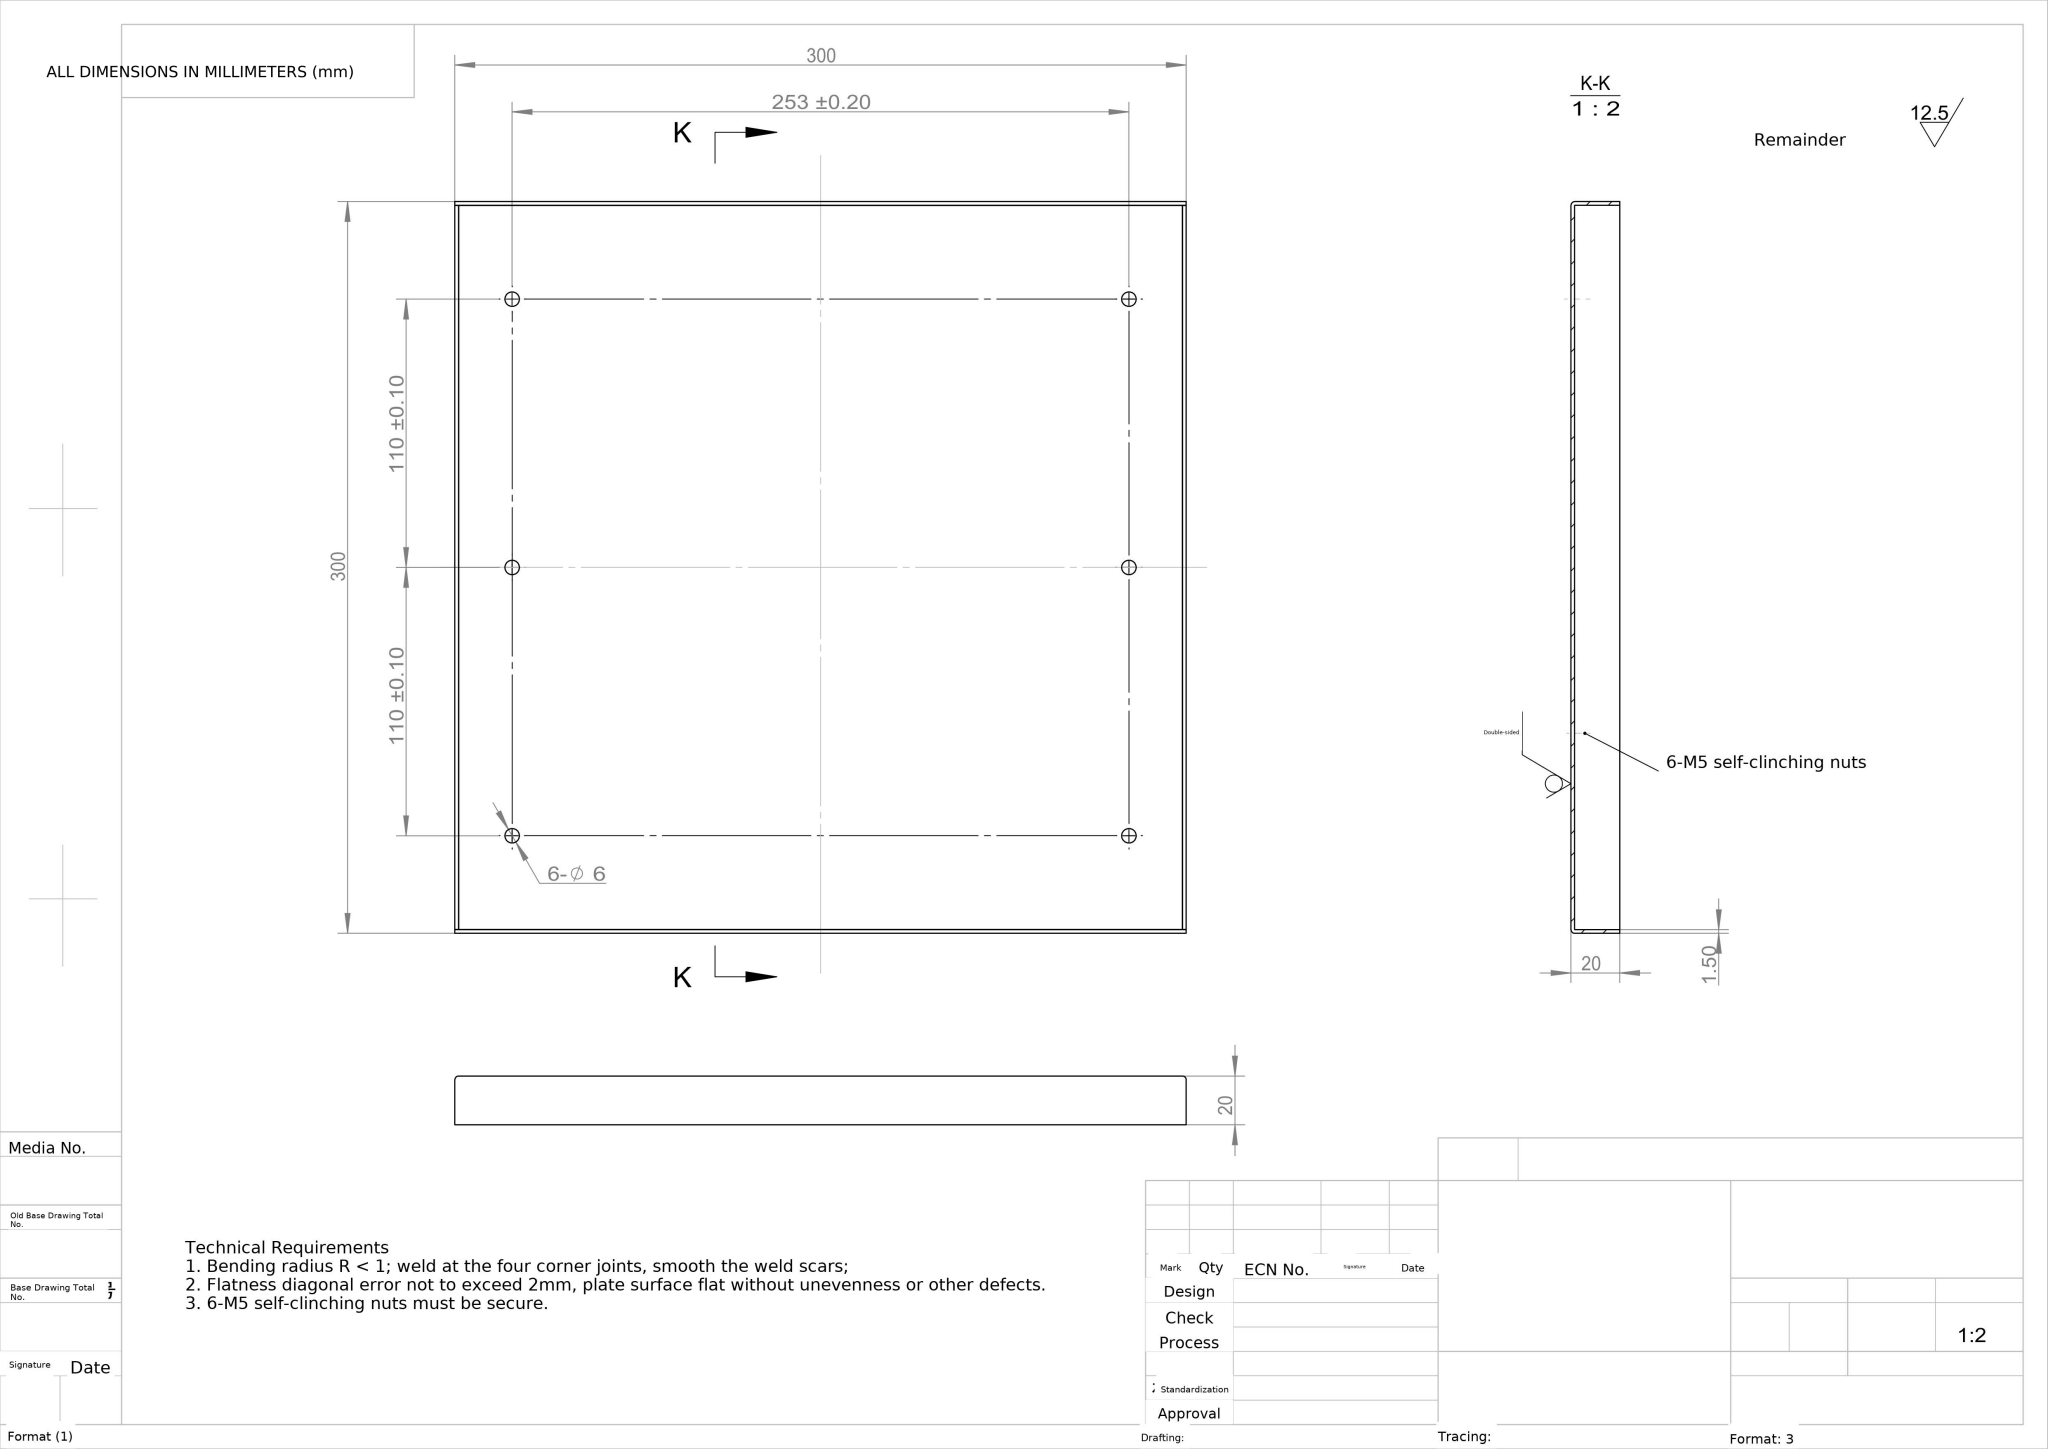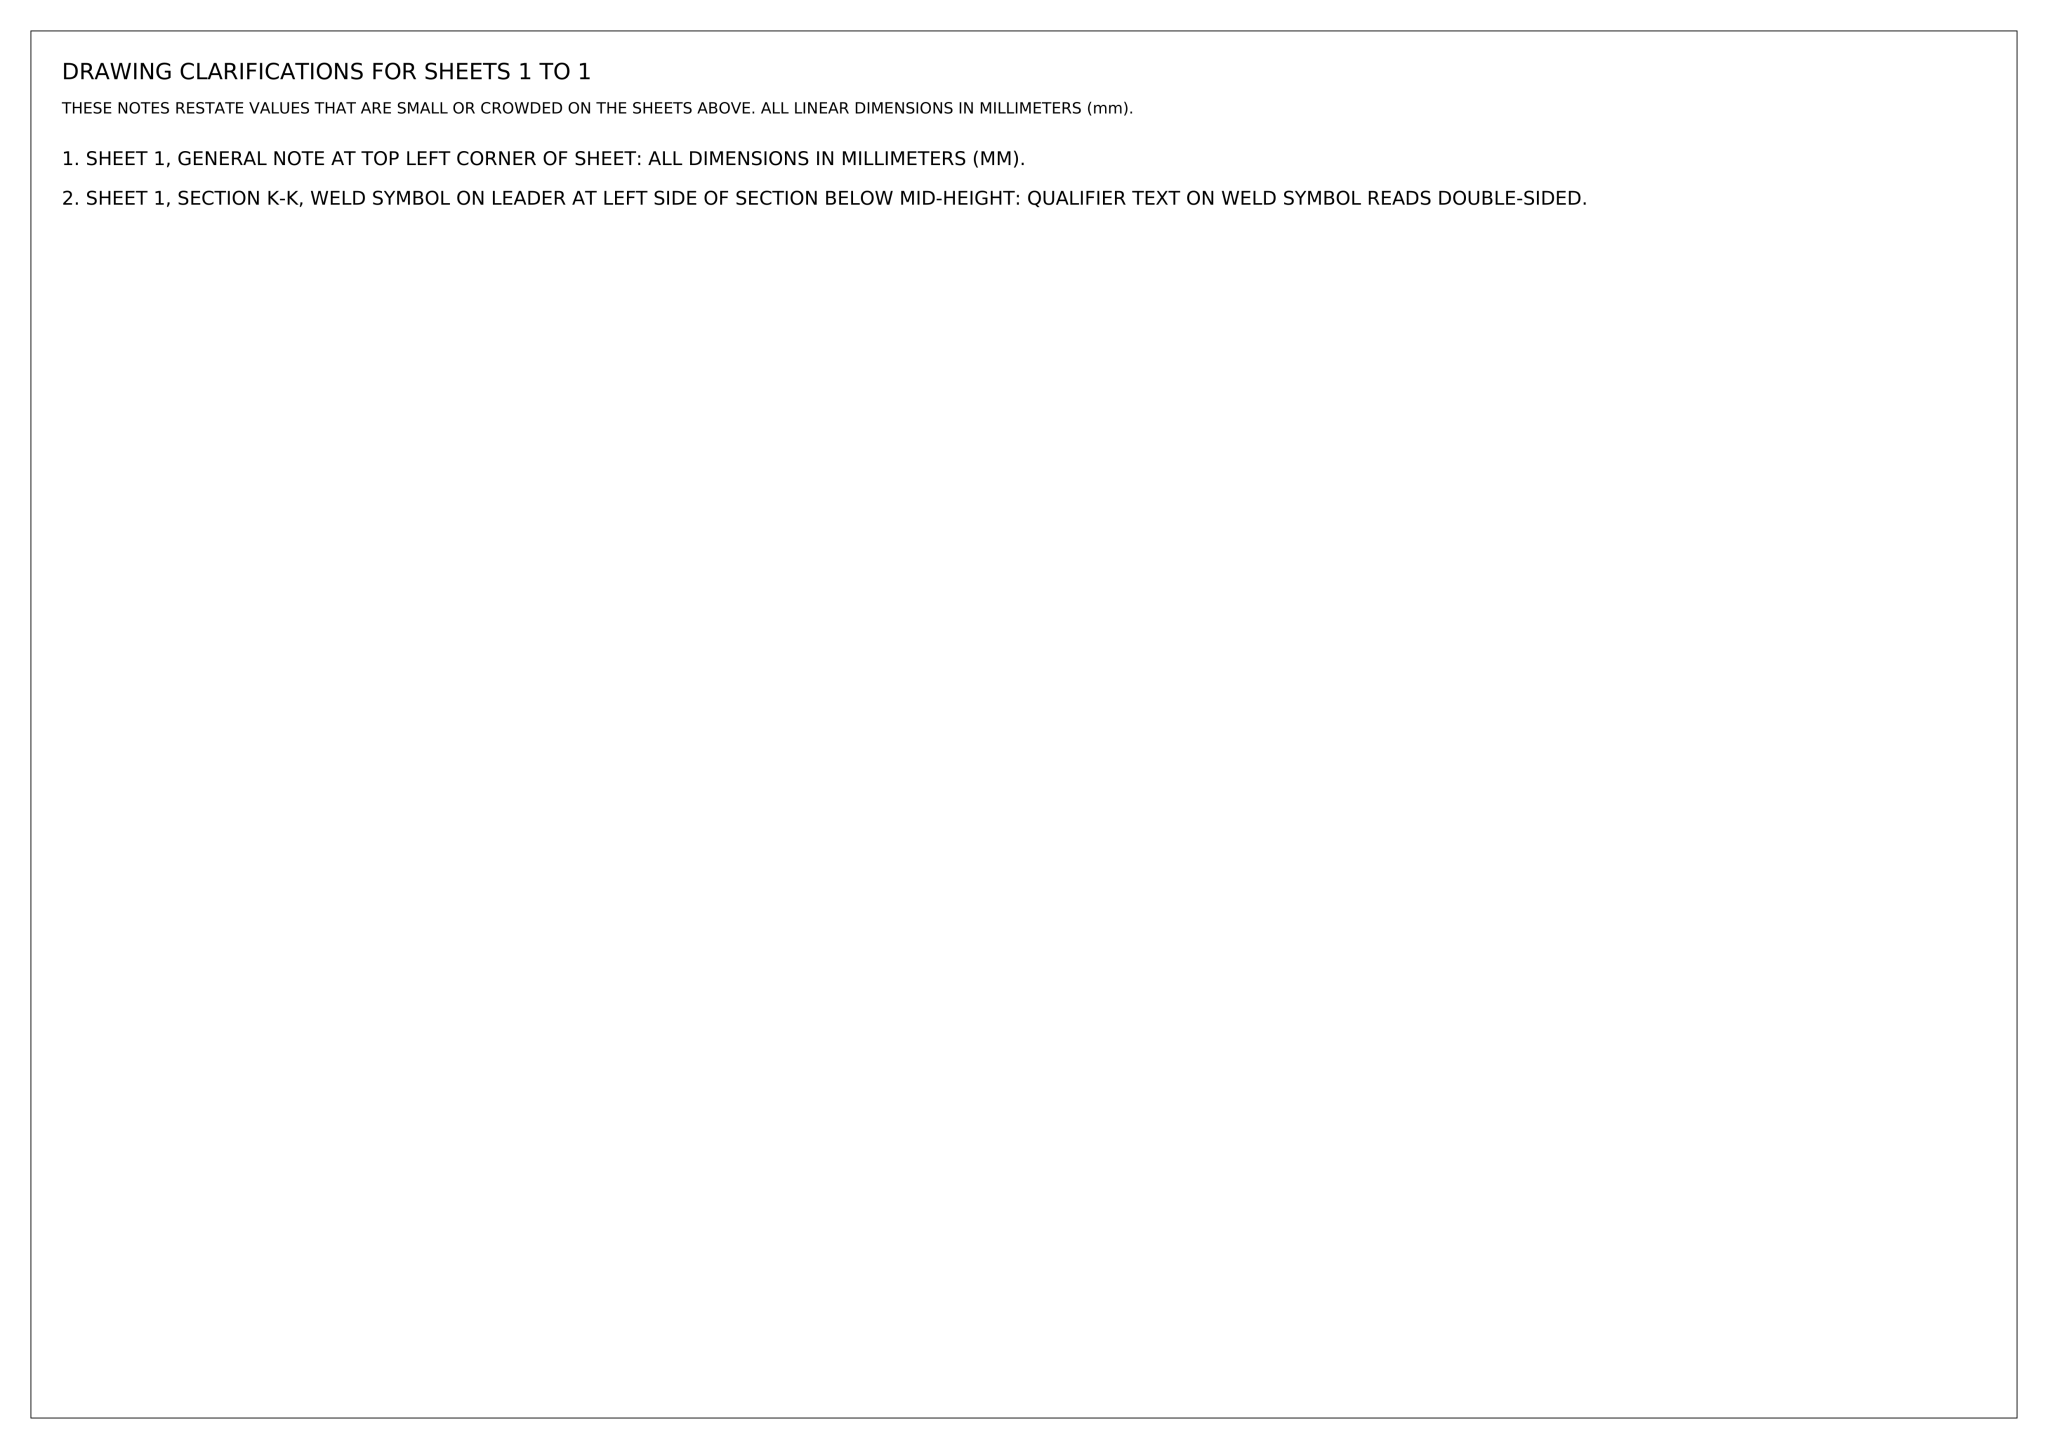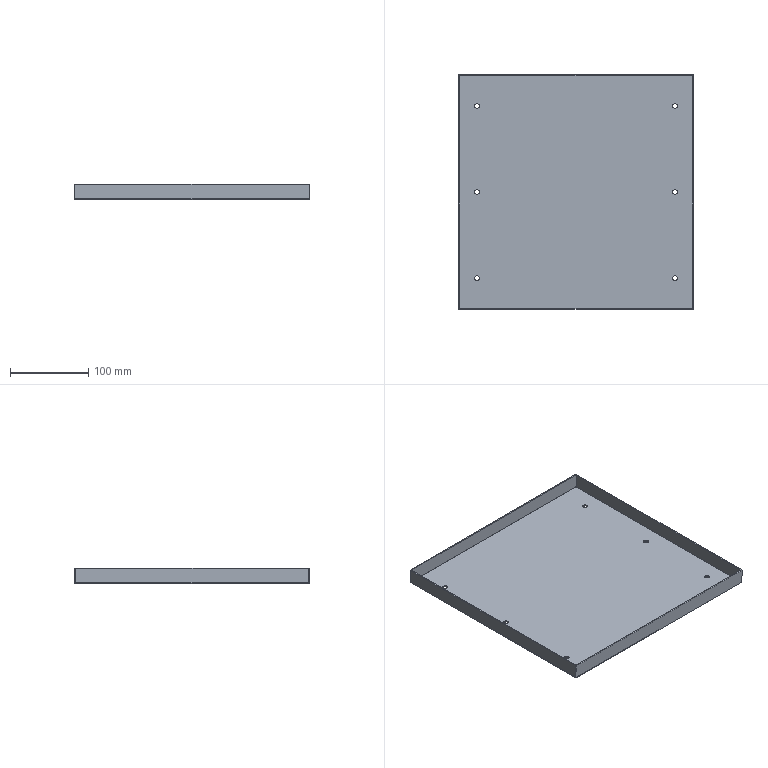Part | NX | mm | 1 solid | 54 faces | box 300 x 300 x 20 mm | volume 167202 mm3 | plane 34 | cylinder 20 | commonest cylinder face diameters 6 x12 3.2 x4 0.2 x4